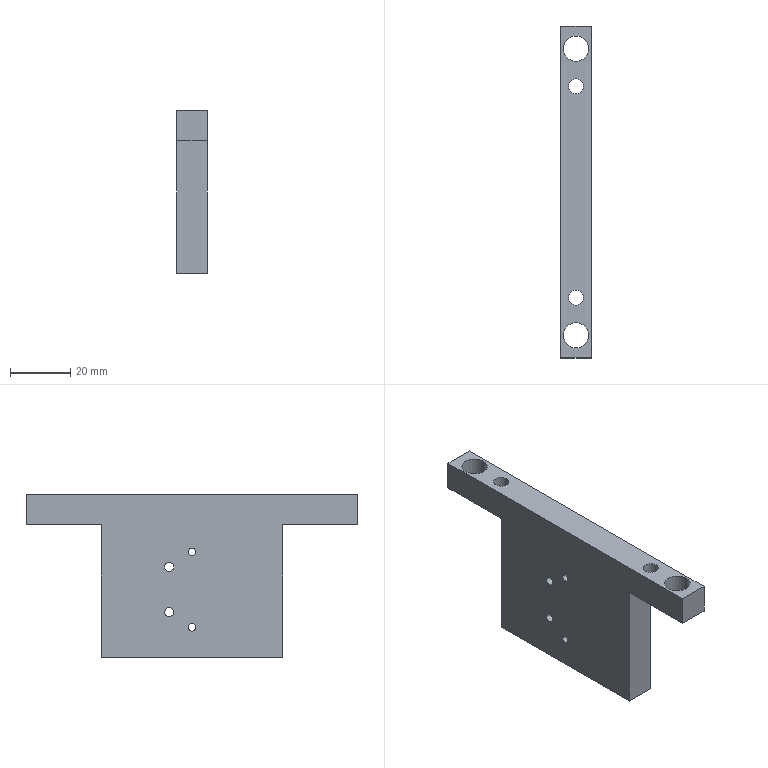Component | SolidWorks | JQ-2-0-002-1 | 1 solid | 34 faces | box 10 x 110 x 54 mm | volume 35051 mm3 | cylinder 20 | plane 10 | cone 4 | commonest cylinder face diameters 5 x8 3 x4 8.4 x4 2.5 x4
STEP:
#1=CARTESIAN_POINT('',(-13.467,1.509,-0.03421));
#2=VERTEX_POINT('',#1);
#3=CARTESIAN_POINT('',(-13.467,1.391,-0.03421));
#4=VERTEX_POINT('',#3);
#5=CARTESIAN_POINT('',(-13.467,1.45,-0.03421));
#6=DIRECTION('',(-1.,0.,0.));
#7=DIRECTION('',(0.,-1.,0.));
#8=AXIS2_PLACEMENT_3D('',#5,#6,#7);
#9=CIRCLE('',#8,0.05906);
#10=EDGE_CURVE('',#2,#4,#9,.T.);
#11=ORIENTED_EDGE('',*,*,#10,.T.);
#12=CARTESIAN_POINT('',(-13.073,1.391,-0.03421));
#13=VERTEX_POINT('',#12);
#14=CARTESIAN_POINT('',(-13.467,1.391,-0.03421));
#15=DIRECTION('',(1.,-0.,-0.));
#16=VECTOR('',#15,39.37);
#17=LINE('',#14,#16);
#18=EDGE_CURVE('',#4,#13,#17,.T.);
#19=ORIENTED_EDGE('',*,*,#18,.T.);
#20=CARTESIAN_POINT('',(-13.073,1.509,-0.03421));
#21=VERTEX_POINT('',#20);
#22=CARTESIAN_POINT('',(-13.073,1.45,-0.03421));
#23=DIRECTION('',(1.,-0.,-0.));
#24=DIRECTION('',(0.,1.,0.));
#25=AXIS2_PLACEMENT_3D('',#22,#23,#24);
#26=CIRCLE('',#25,0.05906);
#27=EDGE_CURVE('',#13,#21,#26,.T.);
#28=ORIENTED_EDGE('',*,*,#27,.T.);
#29=CARTESIAN_POINT('',(-13.467,1.509,-0.03421));
#30=DIRECTION('',(1.,-0.,-0.));
#31=VECTOR('',#30,39.37);
#32=LINE('',#29,#31);
#33=EDGE_CURVE('',#2,#21,#32,.T.);
#34=ORIENTED_EDGE('',*,*,#33,.F.);
#35=EDGE_LOOP('',(#11,#19,#28,#34));
#36=FACE_OUTER_BOUND('',#35,.T.);
#37=CARTESIAN_POINT('',(-13.467,1.45,-0.03421));
#38=DIRECTION('',(1.,-0.,-0.));
#39=DIRECTION('',(0.,1.,0.));
#40=AXIS2_PLACEMENT_3D('',#37,#38,#39);
#41=CYLINDRICAL_SURFACE('',#40,0.05906);
#42=ADVANCED_FACE('',(#36),#41,.F.);
#43=CARTESIAN_POINT('',(-13.467,1.509,0.5563));
#44=VERTEX_POINT('',#43);
#45=CARTESIAN_POINT('',(-13.467,1.391,0.5563));
#46=VERTEX_POINT('',#45);
#47=CARTESIAN_POINT('',(-13.467,1.45,0.5563));
#48=DIRECTION('',(-1.,0.,0.));
#49=DIRECTION('',(0.,-1.,0.));
#50=AXIS2_PLACEMENT_3D('',#47,#48,#49);
#51=CIRCLE('',#50,0.05906);
#52=EDGE_CURVE('',#44,#46,#51,.T.);
#53=ORIENTED_EDGE('',*,*,#52,.T.);
#54=CARTESIAN_POINT('',(-13.073,1.391,0.5563));
#55=VERTEX_POINT('',#54);
#56=CARTESIAN_POINT('',(-13.467,1.391,0.5563));
#57=DIRECTION('',(1.,-0.,-0.));
#58=VECTOR('',#57,39.37);
#59=LINE('',#56,#58);
#60=EDGE_CURVE('',#46,#55,#59,.T.);
#61=ORIENTED_EDGE('',*,*,#60,.T.);
#62=CARTESIAN_POINT('',(-13.073,1.509,0.5563));
#63=VERTEX_POINT('',#62);
#64=CARTESIAN_POINT('',(-13.073,1.45,0.5563));
#65=DIRECTION('',(1.,-0.,-0.));
#66=DIRECTION('',(0.,1.,0.));
#67=AXIS2_PLACEMENT_3D('',#64,#65,#66);
#68=CIRCLE('',#67,0.05906);
#69=EDGE_CURVE('',#55,#63,#68,.T.);
#70=ORIENTED_EDGE('',*,*,#69,.T.);
#71=CARTESIAN_POINT('',(-13.467,1.509,0.5563));
#72=DIRECTION('',(1.,-0.,-0.));
#73=VECTOR('',#72,39.37);
#74=LINE('',#71,#73);
#75=EDGE_CURVE('',#44,#63,#74,.T.);
#76=ORIENTED_EDGE('',*,*,#75,.F.);
#77=EDGE_LOOP('',(#53,#61,#70,#76));
#78=FACE_OUTER_BOUND('',#77,.T.);
#79=CARTESIAN_POINT('',(-13.467,1.45,0.5563));
#80=DIRECTION('',(1.,-0.,-0.));
#81=DIRECTION('',(0.,1.,0.));
#82=AXIS2_PLACEMENT_3D('',#79,#80,#81);
#83=CYLINDRICAL_SURFACE('',#82,0.05906);
#84=ADVANCED_FACE('',(#78),#83,.F.);
#85=CARTESIAN_POINT('',(-13.368,-0.2229,1.108));
#86=VERTEX_POINT('',#85);
#87=CARTESIAN_POINT('',(-13.172,-0.2229,1.108));
#88=VERTEX_POINT('',#87);
#89=CARTESIAN_POINT('',(-13.27,-0.2229,1.108));
#90=DIRECTION('',(0.,-0.,1.));
#91=DIRECTION('',(-1.,0.,0.));
#92=AXIS2_PLACEMENT_3D('',#89,#90,#91);
#93=CIRCLE('',#92,0.09843);
#94=EDGE_CURVE('',#86,#88,#93,.T.);
#95=ORIENTED_EDGE('',*,*,#94,.F.);
#96=CARTESIAN_POINT('',(-13.368,-0.2229,1.501));
#97=VERTEX_POINT('',#96);
#98=CARTESIAN_POINT('',(-13.368,-0.2229,-0.6248));
#99=DIRECTION('',(0.,-0.,1.));
#100=VECTOR('',#99,39.37);
#101=LINE('',#98,#100);
#102=EDGE_CURVE('',#86,#97,#101,.T.);
#103=ORIENTED_EDGE('',*,*,#102,.T.);
#104=CARTESIAN_POINT('',(-13.172,-0.2229,1.501));
#105=VERTEX_POINT('',#104);
#106=CARTESIAN_POINT('',(-13.27,-0.2229,1.501));
#107=DIRECTION('',(0.,-0.,1.));
#108=DIRECTION('',(1.,-0.,0.));
#109=AXIS2_PLACEMENT_3D('',#106,#107,#108);
#110=CIRCLE('',#109,0.09843);
#111=EDGE_CURVE('',#97,#105,#110,.T.);
#112=ORIENTED_EDGE('',*,*,#111,.T.);
#113=CARTESIAN_POINT('',(-13.172,-0.2229,-0.6248));
#114=DIRECTION('',(0.,-0.,1.));
#115=VECTOR('',#114,39.37);
#116=LINE('',#113,#115);
#117=EDGE_CURVE('',#88,#105,#116,.T.);
#118=ORIENTED_EDGE('',*,*,#117,.F.);
#119=EDGE_LOOP('',(#95,#103,#112,#118));
#120=FACE_OUTER_BOUND('',#119,.T.);
#121=CARTESIAN_POINT('',(-13.27,-0.2229,-0.6248));
#122=DIRECTION('',(0.,-0.,1.));
#123=DIRECTION('',(1.,-0.,0.));
#124=AXIS2_PLACEMENT_3D('',#121,#122,#123);
#125=CYLINDRICAL_SURFACE('',#124,0.09843);
#126=ADVANCED_FACE('',(#120),#125,.F.);
#127=CARTESIAN_POINT('',(-13.368,2.533,1.108));
#128=VERTEX_POINT('',#127);
#129=CARTESIAN_POINT('',(-13.172,2.533,1.108));
#130=VERTEX_POINT('',#129);
#131=CARTESIAN_POINT('',(-13.27,2.533,1.108));
#132=DIRECTION('',(0.,-0.,1.));
#133=DIRECTION('',(0.,1.,0.));
#134=AXIS2_PLACEMENT_3D('',#131,#132,#133);
#135=CIRCLE('',#134,0.09843);
#136=EDGE_CURVE('',#128,#130,#135,.T.);
#137=ORIENTED_EDGE('',*,*,#136,.F.);
#138=CARTESIAN_POINT('',(-13.368,2.533,1.501));
#139=VERTEX_POINT('',#138);
#140=CARTESIAN_POINT('',(-13.368,2.533,-0.6248));
#141=DIRECTION('',(0.,-0.,1.));
#142=VECTOR('',#141,39.37);
#143=LINE('',#140,#142);
#144=EDGE_CURVE('',#128,#139,#143,.T.);
#145=ORIENTED_EDGE('',*,*,#144,.T.);
#146=CARTESIAN_POINT('',(-13.172,2.533,1.501));
#147=VERTEX_POINT('',#146);
#148=CARTESIAN_POINT('',(-13.27,2.533,1.501));
#149=DIRECTION('',(0.,-0.,1.));
#150=DIRECTION('',(1.,0.,0.));
#151=AXIS2_PLACEMENT_3D('',#148,#149,#150);
#152=CIRCLE('',#151,0.09843);
#153=EDGE_CURVE('',#139,#147,#152,.T.);
#154=ORIENTED_EDGE('',*,*,#153,.T.);
#155=CARTESIAN_POINT('',(-13.172,2.533,-0.6248));
#156=DIRECTION('',(0.,-0.,1.));
#157=VECTOR('',#156,39.37);
#158=LINE('',#155,#157);
#159=EDGE_CURVE('',#130,#147,#158,.T.);
#160=ORIENTED_EDGE('',*,*,#159,.F.);
#161=EDGE_LOOP('',(#137,#145,#154,#160));
#162=FACE_OUTER_BOUND('',#161,.T.);
#163=CARTESIAN_POINT('',(-13.27,2.533,-0.6248));
#164=DIRECTION('',(0.,-0.,1.));
#165=DIRECTION('',(1.,0.,0.));
#166=AXIS2_PLACEMENT_3D('',#163,#164,#165);
#167=CYLINDRICAL_SURFACE('',#166,0.09843);
#168=ADVANCED_FACE('',(#162),#167,.F.);
#169=CARTESIAN_POINT('',(-13.435,3.025,1.108));
#170=VERTEX_POINT('',#169);
#171=CARTESIAN_POINT('',(-13.105,3.025,1.108));
#172=VERTEX_POINT('',#171);
#173=CARTESIAN_POINT('',(-13.27,3.025,1.108));
#174=DIRECTION('',(0.,-0.,1.));
#175=DIRECTION('',(0.,1.,0.));
#176=AXIS2_PLACEMENT_3D('',#173,#174,#175);
#177=CIRCLE('',#176,0.1654);
#178=EDGE_CURVE('',#170,#172,#177,.T.);
#179=ORIENTED_EDGE('',*,*,#178,.F.);
#180=CARTESIAN_POINT('',(-13.435,3.025,1.501));
#181=VERTEX_POINT('',#180);
#182=CARTESIAN_POINT('',(-13.435,3.025,-0.6248));
#183=DIRECTION('',(0.,-0.,1.));
#184=VECTOR('',#183,39.37);
#185=LINE('',#182,#184);
#186=EDGE_CURVE('',#170,#181,#185,.T.);
#187=ORIENTED_EDGE('',*,*,#186,.T.);
#188=CARTESIAN_POINT('',(-13.105,3.025,1.501));
#189=VERTEX_POINT('',#188);
#190=CARTESIAN_POINT('',(-13.27,3.025,1.501));
#191=DIRECTION('',(0.,-0.,1.));
#192=DIRECTION('',(1.,0.,0.));
#193=AXIS2_PLACEMENT_3D('',#190,#191,#192);
#194=CIRCLE('',#193,0.1654);
#195=EDGE_CURVE('',#181,#189,#194,.T.);
#196=ORIENTED_EDGE('',*,*,#195,.T.);
#197=CARTESIAN_POINT('',(-13.105,3.025,-0.6248));
#198=DIRECTION('',(0.,-0.,1.));
#199=VECTOR('',#198,39.37);
#200=LINE('',#197,#199);
#201=EDGE_CURVE('',#172,#189,#200,.T.);
#202=ORIENTED_EDGE('',*,*,#201,.F.);
#203=EDGE_LOOP('',(#179,#187,#196,#202));
#204=FACE_OUTER_BOUND('',#203,.T.);
#205=CARTESIAN_POINT('',(-13.27,3.025,-0.6248));
#206=DIRECTION('',(0.,-0.,1.));
#207=DIRECTION('',(1.,0.,0.));
#208=AXIS2_PLACEMENT_3D('',#205,#206,#207);
#209=CYLINDRICAL_SURFACE('',#208,0.1654);
#210=ADVANCED_FACE('',(#204),#209,.F.);
#211=CARTESIAN_POINT('',(-13.435,-0.715,1.108));
#212=VERTEX_POINT('',#211);
#213=CARTESIAN_POINT('',(-13.105,-0.715,1.108));
#214=VERTEX_POINT('',#213);
#215=CARTESIAN_POINT('',(-13.27,-0.715,1.108));
#216=DIRECTION('',(0.,-0.,1.));
#217=DIRECTION('',(-1.,0.,0.));
#218=AXIS2_PLACEMENT_3D('',#215,#216,#217);
#219=CIRCLE('',#218,0.1654);
#220=EDGE_CURVE('',#212,#214,#219,.T.);
#221=ORIENTED_EDGE('',*,*,#220,.F.);
#222=CARTESIAN_POINT('',(-13.435,-0.715,1.501));
#223=VERTEX_POINT('',#222);
#224=CARTESIAN_POINT('',(-13.435,-0.715,-0.6248));
#225=DIRECTION('',(0.,-0.,1.));
#226=VECTOR('',#225,39.37);
#227=LINE('',#224,#226);
#228=EDGE_CURVE('',#212,#223,#227,.T.);
#229=ORIENTED_EDGE('',*,*,#228,.T.);
#230=CARTESIAN_POINT('',(-13.105,-0.715,1.501));
#231=VERTEX_POINT('',#230);
#232=CARTESIAN_POINT('',(-13.27,-0.715,1.501));
#233=DIRECTION('',(0.,-0.,1.));
#234=DIRECTION('',(1.,-0.,0.));
#235=AXIS2_PLACEMENT_3D('',#232,#233,#234);
#236=CIRCLE('',#235,0.1654);
#237=EDGE_CURVE('',#223,#231,#236,.T.);
#238=ORIENTED_EDGE('',*,*,#237,.T.);
#239=CARTESIAN_POINT('',(-13.105,-0.715,-0.6248));
#240=DIRECTION('',(0.,-0.,1.));
#241=VECTOR('',#240,39.37);
#242=LINE('',#239,#241);
#243=EDGE_CURVE('',#214,#231,#242,.T.);
#244=ORIENTED_EDGE('',*,*,#243,.F.);
#245=EDGE_LOOP('',(#221,#229,#238,#244));
#246=FACE_OUTER_BOUND('',#245,.T.);
#247=CARTESIAN_POINT('',(-13.27,-0.715,-0.6248));
#248=DIRECTION('',(0.,-0.,1.));
#249=DIRECTION('',(1.,-0.,0.));
#250=AXIS2_PLACEMENT_3D('',#247,#248,#249);
#251=CYLINDRICAL_SURFACE('',#250,0.1654);
#252=ADVANCED_FACE('',(#246),#251,.F.);
#253=CARTESIAN_POINT('',(-13.172,2.139,-0.03421));
#254=VERTEX_POINT('',#253);
#255=CARTESIAN_POINT('',(-13.368,2.139,-0.03421));
#256=VERTEX_POINT('',#255);
#257=CARTESIAN_POINT('',(-13.27,2.139,-0.03421));
#258=DIRECTION('',(-0.,0.,-1.));
#259=DIRECTION('',(-1.,0.,0.));
#260=AXIS2_PLACEMENT_3D('',#257,#258,#259);
#261=CIRCLE('',#260,0.09843);
#262=EDGE_CURVE('',#254,#256,#261,.T.);
#263=ORIENTED_EDGE('',*,*,#262,.F.);
#264=CARTESIAN_POINT('',(-13.172,2.139,-0.6248));
#265=VERTEX_POINT('',#264);
#266=CARTESIAN_POINT('',(-13.172,2.139,-0.6248));
#267=DIRECTION('',(-0.,0.,-1.));
#268=VECTOR('',#267,39.37);
#269=LINE('',#266,#268);
#270=EDGE_CURVE('',#254,#265,#269,.T.);
#271=ORIENTED_EDGE('',*,*,#270,.T.);
#272=CARTESIAN_POINT('',(-13.368,2.139,-0.6248));
#273=VERTEX_POINT('',#272);
#274=CARTESIAN_POINT('',(-13.27,2.139,-0.6248));
#275=DIRECTION('',(-0.,0.,-1.));
#276=DIRECTION('',(-1.,0.,0.));
#277=AXIS2_PLACEMENT_3D('',#274,#275,#276);
#278=CIRCLE('',#277,0.09843);
#279=EDGE_CURVE('',#265,#273,#278,.T.);
#280=ORIENTED_EDGE('',*,*,#279,.T.);
#281=CARTESIAN_POINT('',(-13.368,2.139,-0.6248));
#282=DIRECTION('',(-0.,0.,-1.));
#283=VECTOR('',#282,39.37);
#284=LINE('',#281,#283);
#285=EDGE_CURVE('',#256,#273,#284,.T.);
#286=ORIENTED_EDGE('',*,*,#285,.F.);
#287=EDGE_LOOP('',(#263,#271,#280,#286));
#288=FACE_OUTER_BOUND('',#287,.T.);
#289=CARTESIAN_POINT('',(-13.27,2.139,-0.6248));
#290=DIRECTION('',(-0.,0.,-1.));
#291=DIRECTION('',(-1.,0.,0.));
#292=AXIS2_PLACEMENT_3D('',#289,#290,#291);
#293=CYLINDRICAL_SURFACE('',#292,0.09843);
#294=ADVANCED_FACE('',(#288),#293,.F.);
#295=CARTESIAN_POINT('',(-13.27,2.139,0.02493));
#296=VERTEX_POINT('',#295);
#297=CARTESIAN_POINT('',(-13.368,2.139,-0.03421));
#298=DIRECTION('',(-0.8572,0.,-0.515));
#299=VECTOR('',#298,39.37);
#300=LINE('',#297,#299);
#301=EDGE_CURVE('',#296,#256,#300,.T.);
#302=ORIENTED_EDGE('',*,*,#301,.F.);
#303=CARTESIAN_POINT('',(-13.172,2.139,-0.03421));
#304=DIRECTION('',(0.8572,-0.,-0.515));
#305=VECTOR('',#304,39.37);
#306=LINE('',#303,#305);
#307=EDGE_CURVE('',#296,#254,#306,.T.);
#308=ORIENTED_EDGE('',*,*,#307,.T.);
#309=ORIENTED_EDGE('',*,*,#262,.T.);
#310=EDGE_LOOP('',(#302,#308,#309));
#311=FACE_OUTER_BOUND('',#310,.T.);
#312=CARTESIAN_POINT('',(-13.27,2.139,-0.03421));
#313=DIRECTION('',(-0.,0.,-1.));
#314=DIRECTION('',(-1.,0.,0.));
#315=AXIS2_PLACEMENT_3D('',#312,#313,#314);
#316=CONICAL_SURFACE('',#315,0.09843,1.03);
#317=ADVANCED_FACE('',(#311),#316,.F.);
#318=CARTESIAN_POINT('',(-13.172,0.1708,-0.03421));
#319=VERTEX_POINT('',#318);
#320=CARTESIAN_POINT('',(-13.368,0.1708,-0.03421));
#321=VERTEX_POINT('',#320);
#322=CARTESIAN_POINT('',(-13.27,0.1708,-0.03421));
#323=DIRECTION('',(-0.,0.,-1.));
#324=DIRECTION('',(-1.,0.,0.));
#325=AXIS2_PLACEMENT_3D('',#322,#323,#324);
#326=CIRCLE('',#325,0.09843);
#327=EDGE_CURVE('',#319,#321,#326,.T.);
#328=ORIENTED_EDGE('',*,*,#327,.F.);
#329=CARTESIAN_POINT('',(-13.172,0.1708,-0.6248));
#330=VERTEX_POINT('',#329);
#331=CARTESIAN_POINT('',(-13.172,0.1708,-0.6248));
#332=DIRECTION('',(-0.,0.,-1.));
#333=VECTOR('',#332,39.37);
#334=LINE('',#331,#333);
#335=EDGE_CURVE('',#319,#330,#334,.T.);
#336=ORIENTED_EDGE('',*,*,#335,.T.);
#337=CARTESIAN_POINT('',(-13.368,0.1708,-0.6248));
#338=VERTEX_POINT('',#337);
#339=CARTESIAN_POINT('',(-13.27,0.1708,-0.6248));
#340=DIRECTION('',(-0.,0.,-1.));
#341=DIRECTION('',(-1.,0.,0.));
#342=AXIS2_PLACEMENT_3D('',#339,#340,#341);
#343=CIRCLE('',#342,0.09843);
#344=EDGE_CURVE('',#330,#338,#343,.T.);
#345=ORIENTED_EDGE('',*,*,#344,.T.);
#346=CARTESIAN_POINT('',(-13.368,0.1708,-0.6248));
#347=DIRECTION('',(-0.,0.,-1.));
#348=VECTOR('',#347,39.37);
#349=LINE('',#346,#348);
#350=EDGE_CURVE('',#321,#338,#349,.T.);
#351=ORIENTED_EDGE('',*,*,#350,.F.);
#352=EDGE_LOOP('',(#328,#336,#345,#351));
#353=FACE_OUTER_BOUND('',#352,.T.);
#354=CARTESIAN_POINT('',(-13.27,0.1708,-0.6248));
#355=DIRECTION('',(-0.,0.,-1.));
#356=DIRECTION('',(-1.,0.,0.));
#357=AXIS2_PLACEMENT_3D('',#354,#355,#356);
#358=CYLINDRICAL_SURFACE('',#357,0.09843);
#359=ADVANCED_FACE('',(#353),#358,.F.);
#360=CARTESIAN_POINT('',(-13.27,0.1708,0.02493));
#361=VERTEX_POINT('',#360);
#362=CARTESIAN_POINT('',(-13.368,0.1708,-0.03421));
#363=DIRECTION('',(-0.8572,0.,-0.515));
#364=VECTOR('',#363,39.37);
#365=LINE('',#362,#364);
#366=EDGE_CURVE('',#361,#321,#365,.T.);
#367=ORIENTED_EDGE('',*,*,#366,.F.);
#368=CARTESIAN_POINT('',(-13.172,0.1708,-0.03421));
#369=DIRECTION('',(0.8572,-0.,-0.515));
#370=VECTOR('',#369,39.37);
#371=LINE('',#368,#370);
#372=EDGE_CURVE('',#361,#319,#371,.T.);
#373=ORIENTED_EDGE('',*,*,#372,.T.);
#374=ORIENTED_EDGE('',*,*,#327,.T.);
#375=EDGE_LOOP('',(#367,#373,#374));
#376=FACE_OUTER_BOUND('',#375,.T.);
#377=CARTESIAN_POINT('',(-13.27,0.1708,-0.03421));
#378=DIRECTION('',(-0.,0.,-1.));
#379=DIRECTION('',(-1.,0.,0.));
#380=AXIS2_PLACEMENT_3D('',#377,#378,#379);
#381=CONICAL_SURFACE('',#380,0.09843,1.03);
#382=ADVANCED_FACE('',(#376),#381,.F.);
#383=CARTESIAN_POINT('',(-13.467,1.106,0.7532));
#384=VERTEX_POINT('',#383);
#385=CARTESIAN_POINT('',(-13.467,1.204,0.7532));
#386=VERTEX_POINT('',#385);
#387=CARTESIAN_POINT('',(-13.467,1.155,0.7532));
#388=DIRECTION('',(1.,-0.,-0.));
#389=DIRECTION('',(0.,1.,0.));
#390=AXIS2_PLACEMENT_3D('',#387,#388,#389);
#391=CIRCLE('',#390,0.04921);
#392=EDGE_CURVE('',#384,#386,#391,.T.);
#393=ORIENTED_EDGE('',*,*,#392,.F.);
#394=CARTESIAN_POINT('',(-13.073,1.106,0.7532));
#395=VERTEX_POINT('',#394);
#396=CARTESIAN_POINT('',(-13.073,1.106,0.7532));
#397=DIRECTION('',(1.,-0.,-0.));
#398=VECTOR('',#397,39.37);
#399=LINE('',#396,#398);
#400=EDGE_CURVE('',#384,#395,#399,.T.);
#401=ORIENTED_EDGE('',*,*,#400,.T.);
#402=CARTESIAN_POINT('',(-13.073,1.204,0.7532));
#403=VERTEX_POINT('',#402);
#404=CARTESIAN_POINT('',(-13.073,1.155,0.7532));
#405=DIRECTION('',(1.,-0.,-0.));
#406=DIRECTION('',(0.,1.,0.));
#407=AXIS2_PLACEMENT_3D('',#404,#405,#406);
#408=CIRCLE('',#407,0.04921);
#409=EDGE_CURVE('',#395,#403,#408,.T.);
#410=ORIENTED_EDGE('',*,*,#409,.T.);
#411=CARTESIAN_POINT('',(-13.073,1.204,0.7532));
#412=DIRECTION('',(1.,-0.,-0.));
#413=VECTOR('',#412,39.37);
#414=LINE('',#411,#413);
#415=EDGE_CURVE('',#386,#403,#414,.T.);
#416=ORIENTED_EDGE('',*,*,#415,.F.);
#417=EDGE_LOOP('',(#393,#401,#410,#416));
#418=FACE_OUTER_BOUND('',#417,.T.);
#419=CARTESIAN_POINT('',(-13.073,1.155,0.7532));
#420=DIRECTION('',(1.,-0.,-0.));
#421=DIRECTION('',(0.,1.,0.));
#422=AXIS2_PLACEMENT_3D('',#419,#420,#421);
#423=CYLINDRICAL_SURFACE('',#422,0.04921);
#424=ADVANCED_FACE('',(#418),#423,.F.);
#425=CARTESIAN_POINT('',(-13.467,1.106,-0.2311));
#426=VERTEX_POINT('',#425);
#427=CARTESIAN_POINT('',(-13.467,1.204,-0.2311));
#428=VERTEX_POINT('',#427);
#429=CARTESIAN_POINT('',(-13.467,1.155,-0.2311));
#430=DIRECTION('',(1.,-0.,-0.));
#431=DIRECTION('',(0.,1.,0.));
#432=AXIS2_PLACEMENT_3D('',#429,#430,#431);
#433=CIRCLE('',#432,0.04921);
#434=EDGE_CURVE('',#426,#428,#433,.T.);
#435=ORIENTED_EDGE('',*,*,#434,.F.);
#436=CARTESIAN_POINT('',(-13.073,1.106,-0.2311));
#437=VERTEX_POINT('',#436);
#438=CARTESIAN_POINT('',(-13.073,1.106,-0.2311));
#439=DIRECTION('',(1.,-0.,-0.));
#440=VECTOR('',#439,39.37);
#441=LINE('',#438,#440);
#442=EDGE_CURVE('',#426,#437,#441,.T.);
#443=ORIENTED_EDGE('',*,*,#442,.T.);
#444=CARTESIAN_POINT('',(-13.073,1.204,-0.2311));
#445=VERTEX_POINT('',#444);
#446=CARTESIAN_POINT('',(-13.073,1.155,-0.2311));
#447=DIRECTION('',(1.,-0.,-0.));
#448=DIRECTION('',(0.,1.,0.));
#449=AXIS2_PLACEMENT_3D('',#446,#447,#448);
#450=CIRCLE('',#449,0.04921);
#451=EDGE_CURVE('',#437,#445,#450,.T.);
#452=ORIENTED_EDGE('',*,*,#451,.T.);
#453=CARTESIAN_POINT('',(-13.073,1.204,-0.2311));
#454=DIRECTION('',(1.,-0.,-0.));
#455=VECTOR('',#454,39.37);
#456=LINE('',#453,#455);
#457=EDGE_CURVE('',#428,#445,#456,.T.);
#458=ORIENTED_EDGE('',*,*,#457,.F.);
#459=EDGE_LOOP('',(#435,#443,#452,#458));
#460=FACE_OUTER_BOUND('',#459,.T.);
#461=CARTESIAN_POINT('',(-13.073,1.155,-0.2311));
#462=DIRECTION('',(1.,-0.,-0.));
#463=DIRECTION('',(0.,1.,0.));
#464=AXIS2_PLACEMENT_3D('',#461,#462,#463);
#465=CYLINDRICAL_SURFACE('',#464,0.04921);
#466=ADVANCED_FACE('',(#460),#465,.F.);
#467=CARTESIAN_POINT('',(-13.467,-0.02602,1.108));
#468=VERTEX_POINT('',#467);
#469=CARTESIAN_POINT('',(-13.073,-0.02602,1.108));
#470=VERTEX_POINT('',#469);
#471=CARTESIAN_POINT('',(-14.527,-0.02602,1.108));
#472=DIRECTION('',(1.,-0.,-0.));
#473=VECTOR('',#472,39.37);
#474=LINE('',#471,#473);
#475=EDGE_CURVE('',#468,#470,#474,.T.);
#476=ORIENTED_EDGE('',*,*,#475,.F.);
#477=CARTESIAN_POINT('',(-13.467,-0.02602,-0.6248));
#478=VERTEX_POINT('',#477);
#479=CARTESIAN_POINT('',(-13.467,-0.02602,-0.6248));
#480=DIRECTION('',(-0.,0.,-1.));
#481=VECTOR('',#480,39.37);
#482=LINE('',#479,#481);
#483=EDGE_CURVE('',#468,#478,#482,.T.);
#484=ORIENTED_EDGE('',*,*,#483,.T.);
#485=CARTESIAN_POINT('',(-13.073,-0.02602,-0.6248));
#486=VERTEX_POINT('',#485);
#487=CARTESIAN_POINT('',(-13.073,-0.02602,-0.6248));
#488=DIRECTION('',(-1.,0.,0.));
#489=VECTOR('',#488,39.37);
#490=LINE('',#487,#489);
#491=EDGE_CURVE('',#486,#478,#490,.T.);
#492=ORIENTED_EDGE('',*,*,#491,.F.);
#493=CARTESIAN_POINT('',(-13.073,-0.02602,-0.6248));
#494=DIRECTION('',(-0.,0.,-1.));
#495=VECTOR('',#494,39.37);
#496=LINE('',#493,#495);
#497=EDGE_CURVE('',#470,#486,#496,.T.);
#498=ORIENTED_EDGE('',*,*,#497,.F.);
#499=EDGE_LOOP('',(#476,#484,#492,#498));
#500=FACE_OUTER_BOUND('',#499,.T.);
#501=CARTESIAN_POINT('',(-13.073,-0.02602,-0.6248));
#502=DIRECTION('',(0.,1.,0.));
#503=DIRECTION('',(-1.,0.,0.));
#504=AXIS2_PLACEMENT_3D('',#501,#502,#503);
#505=PLANE('',#504);
#506=ADVANCED_FACE('',(#500),#505,.F.);
#507=CARTESIAN_POINT('',(-13.27,2.139,-0.6248));
#508=DIRECTION('',(-0.,0.,-1.));
#509=DIRECTION('',(-1.,0.,0.));
#510=AXIS2_PLACEMENT_3D('',#507,#508,#509);
#511=CIRCLE('',#510,0.09843);
#512=EDGE_CURVE('',#273,#265,#511,.T.);
#513=ORIENTED_EDGE('',*,*,#512,.F.);
#514=ORIENTED_EDGE('',*,*,#279,.F.);
#515=EDGE_LOOP('',(#513,#514));
#516=FACE_BOUND('',#515,.T.);
#517=CARTESIAN_POINT('',(-13.27,0.1708,-0.6248));
#518=DIRECTION('',(-0.,0.,-1.));
#519=DIRECTION('',(-1.,0.,0.));
#520=AXIS2_PLACEMENT_3D('',#517,#518,#519);
#521=CIRCLE('',#520,0.09843);
#522=EDGE_CURVE('',#338,#330,#521,.T.);
#523=ORIENTED_EDGE('',*,*,#522,.F.);
#524=ORIENTED_EDGE('',*,*,#344,.F.);
#525=EDGE_LOOP('',(#523,#524));
#526=FACE_BOUND('',#525,.T.);
#527=CARTESIAN_POINT('',(-13.467,2.336,-0.6248));
#528=VERTEX_POINT('',#527);
#529=CARTESIAN_POINT('',(-13.467,-0.02602,-0.6248));
#530=DIRECTION('',(0.,1.,0.));
#531=VECTOR('',#530,39.37);
#532=LINE('',#529,#531);
#533=EDGE_CURVE('',#478,#528,#532,.T.);
#534=ORIENTED_EDGE('',*,*,#533,.T.);
#535=CARTESIAN_POINT('',(-13.073,2.336,-0.6248));
#536=VERTEX_POINT('',#535);
#537=CARTESIAN_POINT('',(-13.073,2.336,-0.6248));
#538=DIRECTION('',(-1.,0.,0.));
#539=VECTOR('',#538,39.37);
#540=LINE('',#537,#539);
#541=EDGE_CURVE('',#536,#528,#540,.T.);
#542=ORIENTED_EDGE('',*,*,#541,.F.);
#543=CARTESIAN_POINT('',(-13.073,-0.02602,-0.6248));
#544=DIRECTION('',(0.,1.,0.));
#545=VECTOR('',#544,39.37);
#546=LINE('',#543,#545);
#547=EDGE_CURVE('',#486,#536,#546,.T.);
#548=ORIENTED_EDGE('',*,*,#547,.F.);
#549=ORIENTED_EDGE('',*,*,#491,.T.);
#550=EDGE_LOOP('',(#534,#542,#548,#549));
#551=FACE_OUTER_BOUND('',#550,.T.);
#552=CARTESIAN_POINT('',(-13.073,-0.02602,-0.6248));
#553=DIRECTION('',(0.,-0.,1.));
#554=DIRECTION('',(1.,-0.,-0.));
#555=AXIS2_PLACEMENT_3D('',#552,#553,#554);
#556=PLANE('',#555);
#557=ADVANCED_FACE('',(#516,#526,#551),#556,.F.);
#558=CARTESIAN_POINT('',(-13.467,2.336,1.108));
#559=VERTEX_POINT('',#558);
#560=CARTESIAN_POINT('',(-13.467,2.336,-0.6248));
#561=DIRECTION('',(0.,-0.,1.));
#562=VECTOR('',#561,39.37);
#563=LINE('',#560,#562);
#564=EDGE_CURVE('',#528,#559,#563,.T.);
#565=ORIENTED_EDGE('',*,*,#564,.T.);
#566=CARTESIAN_POINT('',(-13.073,2.336,1.108));
#567=VERTEX_POINT('',#566);
#568=CARTESIAN_POINT('',(-14.527,2.336,1.108));
#569=DIRECTION('',(1.,-0.,-0.));
#570=VECTOR('',#569,39.37);
#571=LINE('',#568,#570);
#572=EDGE_CURVE('',#559,#567,#571,.T.);
#573=ORIENTED_EDGE('',*,*,#572,.T.);
#574=CARTESIAN_POINT('',(-13.073,2.336,-0.6248));
#575=DIRECTION('',(0.,-0.,1.));
#576=VECTOR('',#575,39.37);
#577=LINE('',#574,#576);
#578=EDGE_CURVE('',#536,#567,#577,.T.);
#579=ORIENTED_EDGE('',*,*,#578,.F.);
#580=ORIENTED_EDGE('',*,*,#541,.T.);
#581=EDGE_LOOP('',(#565,#573,#579,#580));
#582=FACE_OUTER_BOUND('',#581,.T.);
#583=CARTESIAN_POINT('',(-13.073,2.336,-0.6248));
#584=DIRECTION('',(-0.,-1.,-0.));
#585=DIRECTION('',(1.,-0.,-0.));
#586=AXIS2_PLACEMENT_3D('',#583,#584,#585);
#587=PLANE('',#586);
#588=ADVANCED_FACE('',(#582),#587,.F.);
#589=CARTESIAN_POINT('',(-13.27,-0.2229,1.501));
#590=DIRECTION('',(0.,-0.,1.));
#591=DIRECTION('',(1.,-0.,0.));
#592=AXIS2_PLACEMENT_3D('',#589,#590,#591);
#593=CIRCLE('',#592,0.09843);
#594=EDGE_CURVE('',#105,#97,#593,.T.);
#595=ORIENTED_EDGE('',*,*,#594,.F.);
#596=ORIENTED_EDGE('',*,*,#111,.F.);
#597=EDGE_LOOP('',(#595,#596));
#598=FACE_BOUND('',#597,.T.);
#599=CARTESIAN_POINT('',(-13.27,2.533,1.501));
#600=DIRECTION('',(0.,-0.,1.));
#601=DIRECTION('',(1.,0.,0.));
#602=AXIS2_PLACEMENT_3D('',#599,#600,#601);
#603=CIRCLE('',#602,0.09843);
#604=EDGE_CURVE('',#147,#139,#603,.T.);
#605=ORIENTED_EDGE('',*,*,#604,.F.);
#606=ORIENTED_EDGE('',*,*,#153,.F.);
#607=EDGE_LOOP('',(#605,#606));
#608=FACE_BOUND('',#607,.T.);
#609=CARTESIAN_POINT('',(-13.27,3.025,1.501));
#610=DIRECTION('',(0.,-0.,1.));
#611=DIRECTION('',(1.,0.,0.));
#612=AXIS2_PLACEMENT_3D('',#609,#610,#611);
#613=CIRCLE('',#612,0.1654);
#614=EDGE_CURVE('',#189,#181,#613,.T.);
#615=ORIENTED_EDGE('',*,*,#614,.F.);
#616=ORIENTED_EDGE('',*,*,#195,.F.);
#617=EDGE_LOOP('',(#615,#616));
#618=FACE_BOUND('',#617,.T.);
#619=CARTESIAN_POINT('',(-13.27,-0.715,1.501));
#620=DIRECTION('',(0.,-0.,1.));
#621=DIRECTION('',(1.,-0.,0.));
#622=AXIS2_PLACEMENT_3D('',#619,#620,#621);
#623=CIRCLE('',#622,0.1654);
#624=EDGE_CURVE('',#231,#223,#623,.T.);
#625=ORIENTED_EDGE('',*,*,#624,.F.);
#626=ORIENTED_EDGE('',*,*,#237,.F.);
#627=EDGE_LOOP('',(#625,#626));
#628=FACE_BOUND('',#627,.T.);
#629=CARTESIAN_POINT('',(-13.467,3.32,1.501));
#630=VERTEX_POINT('',#629);
#631=CARTESIAN_POINT('',(-13.467,-1.01,1.501));
#632=VERTEX_POINT('',#631);
#633=CARTESIAN_POINT('',(-13.467,-0.02602,1.501));
#634=DIRECTION('',(-0.,-1.,-0.));
#635=VECTOR('',#634,39.37);
#636=LINE('',#633,#635);
#637=EDGE_CURVE('',#630,#632,#636,.T.);
#638=ORIENTED_EDGE('',*,*,#637,.T.);
#639=CARTESIAN_POINT('',(-13.073,-1.01,1.501));
#640=VERTEX_POINT('',#639);
#641=CARTESIAN_POINT('',(-14.527,-1.01,1.501));
#642=DIRECTION('',(1.,-0.,-0.));
#643=VECTOR('',#642,39.37);
#644=LINE('',#641,#643);
#645=EDGE_CURVE('',#632,#640,#644,.T.);
#646=ORIENTED_EDGE('',*,*,#645,.T.);
#647=CARTESIAN_POINT('',(-13.073,3.32,1.501));
#648=VERTEX_POINT('',#647);
#649=CARTESIAN_POINT('',(-13.073,-0.02602,1.501));
#650=DIRECTION('',(-0.,-1.,-0.));
#651=VECTOR('',#650,39.37);
#652=LINE('',#649,#651);
#653=EDGE_CURVE('',#648,#640,#652,.T.);
#654=ORIENTED_EDGE('',*,*,#653,.F.);
#655=CARTESIAN_POINT('',(-14.527,3.32,1.501));
#656=DIRECTION('',(1.,-0.,-0.));
#657=VECTOR('',#656,39.37);
#658=LINE('',#655,#657);
#659=EDGE_CURVE('',#630,#648,#658,.T.);
#660=ORIENTED_EDGE('',*,*,#659,.F.);
#661=EDGE_LOOP('',(#638,#646,#654,#660));
#662=FACE_OUTER_BOUND('',#661,.T.);
#663=CARTESIAN_POINT('',(-13.073,-0.02602,1.501));
#664=DIRECTION('',(-0.,0.,-1.));
#665=DIRECTION('',(-1.,0.,0.));
#666=AXIS2_PLACEMENT_3D('',#663,#664,#665);
#667=PLANE('',#666);
#668=ADVANCED_FACE('',(#598,#608,#618,#628,#662),#667,.F.);
#669=CARTESIAN_POINT('',(-13.073,1.45,-0.03421));
#670=DIRECTION('',(1.,-0.,-0.));
#671=DIRECTION('',(0.,1.,0.));
#672=AXIS2_PLACEMENT_3D('',#669,#670,#671);
#673=CIRCLE('',#672,0.05906);
#674=EDGE_CURVE('',#21,#13,#673,.T.);
#675=ORIENTED_EDGE('',*,*,#674,.F.);
#676=ORIENTED_EDGE('',*,*,#27,.F.);
#677=EDGE_LOOP('',(#675,#676));
#678=FACE_BOUND('',#677,.T.);
#679=CARTESIAN_POINT('',(-13.073,1.45,0.5563));
#680=DIRECTION('',(1.,-0.,-0.));
#681=DIRECTION('',(0.,1.,0.));
#682=AXIS2_PLACEMENT_3D('',#679,#680,#681);
#683=CIRCLE('',#682,0.05906);
#684=EDGE_CURVE('',#63,#55,#683,.T.);
#685=ORIENTED_EDGE('',*,*,#684,.F.);
#686=ORIENTED_EDGE('',*,*,#69,.F.);
#687=EDGE_LOOP('',(#685,#686));
#688=FACE_BOUND('',#687,.T.);
#689=CARTESIAN_POINT('',(-13.073,1.155,0.7532));
#690=DIRECTION('',(1.,-0.,-0.));
#691=DIRECTION('',(0.,1.,0.));
#692=AXIS2_PLACEMENT_3D('',#689,#690,#691);
#693=CIRCLE('',#692,0.04921);
#694=EDGE_CURVE('',#403,#395,#693,.T.);
#695=ORIENTED_EDGE('',*,*,#694,.F.);
#696=ORIENTED_EDGE('',*,*,#409,.F.);
#697=EDGE_LOOP('',(#695,#696));
#698=FACE_BOUND('',#697,.T.);
#699=CARTESIAN_POINT('',(-13.073,1.155,-0.2311));
#700=DIRECTION('',(1.,-0.,-0.));
#701=DIRECTION('',(0.,1.,0.));
#702=AXIS2_PLACEMENT_3D('',#699,#700,#701);
#703=CIRCLE('',#702,0.04921);
#704=EDGE_CURVE('',#445,#437,#703,.T.);
#705=ORIENTED_EDGE('',*,*,#704,.F.);
#706=ORIENTED_EDGE('',*,*,#451,.F.);
#707=EDGE_LOOP('',(#705,#706));
#708=FACE_BOUND('',#707,.T.);
#709=ORIENTED_EDGE('',*,*,#653,.T.);
#710=CARTESIAN_POINT('',(-13.073,-1.01,1.108));
#711=VERTEX_POINT('',#710);
#712=CARTESIAN_POINT('',(-13.073,-1.01,1.501));
#713=DIRECTION('',(-0.,0.,-1.));
#714=VECTOR('',#713,39.37);
#715=LINE('',#712,#714);
#716=EDGE_CURVE('',#640,#711,#715,.T.);
#717=ORIENTED_EDGE('',*,*,#716,.T.);
#718=CARTESIAN_POINT('',(-13.073,-0.02602,1.108));
#719=DIRECTION('',(0.,1.,0.));
#720=VECTOR('',#719,39.37);
#721=LINE('',#718,#720);
#722=EDGE_CURVE('',#711,#470,#721,.T.);
#723=ORIENTED_EDGE('',*,*,#722,.T.);
#724=ORIENTED_EDGE('',*,*,#497,.T.);
#725=ORIENTED_EDGE('',*,*,#547,.T.);
#726=ORIENTED_EDGE('',*,*,#578,.T.);
#727=CARTESIAN_POINT('',(-13.073,3.32,1.108));
#728=VERTEX_POINT('',#727);
#729=CARTESIAN_POINT('',(-13.073,2.336,1.108));
#730=DIRECTION('',(0.,1.,0.));
#731=VECTOR('',#730,39.37);
#732=LINE('',#729,#731);
#733=EDGE_CURVE('',#567,#728,#732,.T.);
#734=ORIENTED_EDGE('',*,*,#733,.T.);
#735=CARTESIAN_POINT('',(-13.073,3.32,1.501));
#736=DIRECTION('',(0.,0.,1.));
#737=VECTOR('',#736,39.37);
#738=LINE('',#735,#737);
#739=EDGE_CURVE('',#728,#648,#738,.T.);
#740=ORIENTED_EDGE('',*,*,#739,.T.);
#741=EDGE_LOOP('',(#709,#717,#723,#724,#725,#726,#734,#740));
#742=FACE_OUTER_BOUND('',#741,.T.);
#743=CARTESIAN_POINT('',(-13.073,-0.02602,1.501));
#744=DIRECTION('',(-1.,0.,0.));
#745=DIRECTION('',(-0.,-1.,-0.));
#746=AXIS2_PLACEMENT_3D('',#743,#744,#745);
#747=PLANE('',#746);
#748=ADVANCED_FACE('',(#678,#688,#698,#708,#742),#747,.F.);
#749=ORIENTED_EDGE('',*,*,#10,.F.);
#750=CARTESIAN_POINT('',(-13.467,1.45,-0.03421));
#751=DIRECTION('',(-1.,0.,0.));
#752=DIRECTION('',(0.,-1.,0.));
#753=AXIS2_PLACEMENT_3D('',#750,#751,#752);
#754=CIRCLE('',#753,0.05906);
#755=EDGE_CURVE('',#4,#2,#754,.T.);
#756=ORIENTED_EDGE('',*,*,#755,.F.);
#757=EDGE_LOOP('',(#749,#756));
#758=FACE_BOUND('',#757,.T.);
#759=ORIENTED_EDGE('',*,*,#52,.F.);
#760=CARTESIAN_POINT('',(-13.467,1.45,0.5563));
#761=DIRECTION('',(-1.,0.,0.));
#762=DIRECTION('',(0.,-1.,0.));
#763=AXIS2_PLACEMENT_3D('',#760,#761,#762);
#764=CIRCLE('',#763,0.05906);
#765=EDGE_CURVE('',#46,#44,#764,.T.);
#766=ORIENTED_EDGE('',*,*,#765,.F.);
#767=EDGE_LOOP('',(#759,#766));
#768=FACE_BOUND('',#767,.T.);
#769=CARTESIAN_POINT('',(-13.467,1.155,0.7532));
#770=DIRECTION('',(1.,-0.,-0.));
#771=DIRECTION('',(0.,1.,0.));
#772=AXIS2_PLACEMENT_3D('',#769,#770,#771);
#773=CIRCLE('',#772,0.04921);
#774=EDGE_CURVE('',#386,#384,#773,.T.);
#775=ORIENTED_EDGE('',*,*,#774,.T.);
#776=ORIENTED_EDGE('',*,*,#392,.T.);
#777=EDGE_LOOP('',(#775,#776));
#778=FACE_BOUND('',#777,.T.);
#779=CARTESIAN_POINT('',(-13.467,1.155,-0.2311));
#780=DIRECTION('',(1.,-0.,-0.));
#781=DIRECTION('',(0.,1.,0.));
#782=AXIS2_PLACEMENT_3D('',#779,#780,#781);
#783=CIRCLE('',#782,0.04921);
#784=EDGE_CURVE('',#428,#426,#783,.T.);
#785=ORIENTED_EDGE('',*,*,#784,.T.);
#786=ORIENTED_EDGE('',*,*,#434,.T.);
#787=EDGE_LOOP('',(#785,#786));
#788=FACE_BOUND('',#787,.T.);
#789=ORIENTED_EDGE('',*,*,#483,.F.);
#790=CARTESIAN_POINT('',(-13.467,-1.01,1.108));
#791=VERTEX_POINT('',#790);
#792=CARTESIAN_POINT('',(-13.467,-0.02602,1.108));
#793=DIRECTION('',(0.,1.,0.));
#794=VECTOR('',#793,39.37);
#795=LINE('',#792,#794);
#796=EDGE_CURVE('',#791,#468,#795,.T.);
#797=ORIENTED_EDGE('',*,*,#796,.F.);
#798=CARTESIAN_POINT('',(-13.467,-1.01,1.501));
#799=DIRECTION('',(-0.,0.,-1.));
#800=VECTOR('',#799,39.37);
#801=LINE('',#798,#800);
#802=EDGE_CURVE('',#632,#791,#801,.T.);
#803=ORIENTED_EDGE('',*,*,#802,.F.);
#804=ORIENTED_EDGE('',*,*,#637,.F.);
#805=CARTESIAN_POINT('',(-13.467,3.32,1.108));
#806=VERTEX_POINT('',#805);
#807=CARTESIAN_POINT('',(-13.467,3.32,1.501));
#808=DIRECTION('',(0.,0.,1.));
#809=VECTOR('',#808,39.37);
#810=LINE('',#807,#809);
#811=EDGE_CURVE('',#806,#630,#810,.T.);
#812=ORIENTED_EDGE('',*,*,#811,.F.);
#813=CARTESIAN_POINT('',(-13.467,2.336,1.108));
#814=DIRECTION('',(0.,1.,0.));
#815=VECTOR('',#814,39.37);
#816=LINE('',#813,#815);
#817=EDGE_CURVE('',#559,#806,#816,.T.);
#818=ORIENTED_EDGE('',*,*,#817,.F.);
#819=ORIENTED_EDGE('',*,*,#564,.F.);
#820=ORIENTED_EDGE('',*,*,#533,.F.);
#821=EDGE_LOOP('',(#789,#797,#803,#804,#812,#818,#819,#820));
#822=FACE_OUTER_BOUND('',#821,.T.);
#823=CARTESIAN_POINT('',(-13.467,-0.02602,1.501));
#824=DIRECTION('',(-1.,0.,0.));
#825=DIRECTION('',(-0.,-1.,-0.));
#826=AXIS2_PLACEMENT_3D('',#823,#824,#825);
#827=PLANE('',#826);
#828=ADVANCED_FACE('',(#758,#768,#778,#788,#822),#827,.T.);
#829=ORIENTED_EDGE('',*,*,#442,.F.);
#830=ORIENTED_EDGE('',*,*,#784,.F.);
#831=ORIENTED_EDGE('',*,*,#457,.T.);
#832=ORIENTED_EDGE('',*,*,#704,.T.);
#833=EDGE_LOOP('',(#829,#830,#831,#832));
#834=FACE_OUTER_BOUND('',#833,.T.);
#835=CARTESIAN_POINT('',(-13.073,1.155,-0.2311));
#836=DIRECTION('',(1.,-0.,-0.));
#837=DIRECTION('',(0.,1.,0.));
#838=AXIS2_PLACEMENT_3D('',#835,#836,#837);
#839=CYLINDRICAL_SURFACE('',#838,0.04921);
#840=ADVANCED_FACE('',(#834),#839,.F.);
#841=ORIENTED_EDGE('',*,*,#400,.F.);
#842=ORIENTED_EDGE('',*,*,#774,.F.);
#843=ORIENTED_EDGE('',*,*,#415,.T.);
#844=ORIENTED_EDGE('',*,*,#694,.T.);
#845=EDGE_LOOP('',(#841,#842,#843,#844));
#846=FACE_OUTER_BOUND('',#845,.T.);
#847=CARTESIAN_POINT('',(-13.073,1.155,0.7532));
#848=DIRECTION('',(1.,-0.,-0.));
#849=DIRECTION('',(0.,1.,0.));
#850=AXIS2_PLACEMENT_3D('',#847,#848,#849);
#851=CYLINDRICAL_SURFACE('',#850,0.04921);
#852=ADVANCED_FACE('',(#846),#851,.F.);
#853=ORIENTED_EDGE('',*,*,#372,.F.);
#854=ORIENTED_EDGE('',*,*,#366,.T.);
#855=CARTESIAN_POINT('',(-13.27,0.1708,-0.03421));
#856=DIRECTION('',(-0.,0.,-1.));
#857=DIRECTION('',(-1.,0.,0.));
#858=AXIS2_PLACEMENT_3D('',#855,#856,#857);
#859=CIRCLE('',#858,0.09843);
#860=EDGE_CURVE('',#321,#319,#859,.T.);
#861=ORIENTED_EDGE('',*,*,#860,.T.);
#862=EDGE_LOOP('',(#853,#854,#861));
#863=FACE_OUTER_BOUND('',#862,.T.);
#864=CARTESIAN_POINT('',(-13.27,0.1708,-0.03421));
#865=DIRECTION('',(-0.,0.,-1.));
#866=DIRECTION('',(-1.,0.,0.));
#867=AXIS2_PLACEMENT_3D('',#864,#865,#866);
#868=CONICAL_SURFACE('',#867,0.09843,1.03);
#869=ADVANCED_FACE('',(#863),#868,.F.);
#870=ORIENTED_EDGE('',*,*,#335,.F.);
#871=ORIENTED_EDGE('',*,*,#860,.F.);
#872=ORIENTED_EDGE('',*,*,#350,.T.);
#873=ORIENTED_EDGE('',*,*,#522,.T.);
#874=EDGE_LOOP('',(#870,#871,#872,#873));
#875=FACE_OUTER_BOUND('',#874,.T.);
#876=CARTESIAN_POINT('',(-13.27,0.1708,-0.6248));
#877=DIRECTION('',(-0.,0.,-1.));
#878=DIRECTION('',(-1.,0.,0.));
#879=AXIS2_PLACEMENT_3D('',#876,#877,#878);
#880=CYLINDRICAL_SURFACE('',#879,0.09843);
#881=ADVANCED_FACE('',(#875),#880,.F.);
#882=ORIENTED_EDGE('',*,*,#307,.F.);
#883=ORIENTED_EDGE('',*,*,#301,.T.);
#884=CARTESIAN_POINT('',(-13.27,2.139,-0.03421));
#885=DIRECTION('',(-0.,0.,-1.));
#886=DIRECTION('',(-1.,0.,0.));
#887=AXIS2_PLACEMENT_3D('',#884,#885,#886);
#888=CIRCLE('',#887,0.09843);
#889=EDGE_CURVE('',#256,#254,#888,.T.);
#890=ORIENTED_EDGE('',*,*,#889,.T.);
#891=EDGE_LOOP('',(#882,#883,#890));
#892=FACE_OUTER_BOUND('',#891,.T.);
#893=CARTESIAN_POINT('',(-13.27,2.139,-0.03421));
#894=DIRECTION('',(-0.,0.,-1.));
#895=DIRECTION('',(-1.,0.,0.));
#896=AXIS2_PLACEMENT_3D('',#893,#894,#895);
#897=CONICAL_SURFACE('',#896,0.09843,1.03);
#898=ADVANCED_FACE('',(#892),#897,.F.);
#899=ORIENTED_EDGE('',*,*,#270,.F.);
#900=ORIENTED_EDGE('',*,*,#889,.F.);
#901=ORIENTED_EDGE('',*,*,#285,.T.);
#902=ORIENTED_EDGE('',*,*,#512,.T.);
#903=EDGE_LOOP('',(#899,#900,#901,#902));
#904=FACE_OUTER_BOUND('',#903,.T.);
#905=CARTESIAN_POINT('',(-13.27,2.139,-0.6248));
#906=DIRECTION('',(-0.,0.,-1.));
#907=DIRECTION('',(-1.,0.,0.));
#908=AXIS2_PLACEMENT_3D('',#905,#906,#907);
#909=CYLINDRICAL_SURFACE('',#908,0.09843);
#910=ADVANCED_FACE('',(#904),#909,.F.);
#911=ORIENTED_EDGE('',*,*,#645,.F.);
#912=ORIENTED_EDGE('',*,*,#802,.T.);
#913=CARTESIAN_POINT('',(-14.527,-1.01,1.108));
#914=DIRECTION('',(1.,-0.,-0.));
#915=VECTOR('',#914,39.37);
#916=LINE('',#913,#915);
#917=EDGE_CURVE('',#791,#711,#916,.T.);
#918=ORIENTED_EDGE('',*,*,#917,.T.);
#919=ORIENTED_EDGE('',*,*,#716,.F.);
#920=EDGE_LOOP('',(#911,#912,#918,#919));
#921=FACE_OUTER_BOUND('',#920,.T.);
#922=CARTESIAN_POINT('',(-14.527,-1.01,1.501));
#923=DIRECTION('',(-0.,-1.,-0.));
#924=DIRECTION('',(1.,-0.,-0.));
#925=AXIS2_PLACEMENT_3D('',#922,#923,#924);
#926=PLANE('',#925);
#927=ADVANCED_FACE('',(#921),#926,.T.);
#928=CARTESIAN_POINT('',(-13.27,-0.2229,1.108));
#929=DIRECTION('',(0.,-0.,1.));
#930=DIRECTION('',(-1.,0.,0.));
#931=AXIS2_PLACEMENT_3D('',#928,#929,#930);
#932=CIRCLE('',#931,0.09843);
#933=EDGE_CURVE('',#88,#86,#932,.T.);
#934=ORIENTED_EDGE('',*,*,#933,.T.);
#935=ORIENTED_EDGE('',*,*,#94,.T.);
#936=EDGE_LOOP('',(#934,#935));
#937=FACE_BOUND('',#936,.T.);
#938=CARTESIAN_POINT('',(-13.27,-0.715,1.108));
#939=DIRECTION('',(0.,-0.,1.));
#940=DIRECTION('',(-1.,0.,0.));
#941=AXIS2_PLACEMENT_3D('',#938,#939,#940);
#942=CIRCLE('',#941,0.1654);
#943=EDGE_CURVE('',#214,#212,#942,.T.);
#944=ORIENTED_EDGE('',*,*,#943,.T.);
#945=ORIENTED_EDGE('',*,*,#220,.T.);
#946=EDGE_LOOP('',(#944,#945));
#947=FACE_BOUND('',#946,.T.);
#948=ORIENTED_EDGE('',*,*,#917,.F.);
#949=ORIENTED_EDGE('',*,*,#796,.T.);
#950=ORIENTED_EDGE('',*,*,#475,.T.);
#951=ORIENTED_EDGE('',*,*,#722,.F.);
#952=EDGE_LOOP('',(#948,#949,#950,#951));
#953=FACE_OUTER_BOUND('',#952,.T.);
#954=CARTESIAN_POINT('',(-14.527,-0.02602,1.108));
#955=DIRECTION('',(-0.,0.,-1.));
#956=DIRECTION('',(-1.,0.,0.));
#957=AXIS2_PLACEMENT_3D('',#954,#955,#956);
#958=PLANE('',#957);
#959=ADVANCED_FACE('',(#937,#947,#953),#958,.T.);
#960=CARTESIAN_POINT('',(-13.27,2.533,1.108));
#961=DIRECTION('',(0.,-0.,1.));
#962=DIRECTION('',(0.,1.,0.));
#963=AXIS2_PLACEMENT_3D('',#960,#961,#962);
#964=CIRCLE('',#963,0.09843);
#965=EDGE_CURVE('',#130,#128,#964,.T.);
#966=ORIENTED_EDGE('',*,*,#965,.T.);
#967=ORIENTED_EDGE('',*,*,#136,.T.);
#968=EDGE_LOOP('',(#966,#967));
#969=FACE_BOUND('',#968,.T.);
#970=CARTESIAN_POINT('',(-13.27,3.025,1.108));
#971=DIRECTION('',(0.,-0.,1.));
#972=DIRECTION('',(0.,1.,0.));
#973=AXIS2_PLACEMENT_3D('',#970,#971,#972);
#974=CIRCLE('',#973,0.1654);
#975=EDGE_CURVE('',#172,#170,#974,.T.);
#976=ORIENTED_EDGE('',*,*,#975,.T.);
#977=ORIENTED_EDGE('',*,*,#178,.T.);
#978=EDGE_LOOP('',(#976,#977));
#979=FACE_BOUND('',#978,.T.);
#980=ORIENTED_EDGE('',*,*,#572,.F.);
#981=ORIENTED_EDGE('',*,*,#817,.T.);
#982=CARTESIAN_POINT('',(-14.527,3.32,1.108));
#983=DIRECTION('',(1.,-0.,-0.));
#984=VECTOR('',#983,39.37);
#985=LINE('',#982,#984);
#986=EDGE_CURVE('',#806,#728,#985,.T.);
#987=ORIENTED_EDGE('',*,*,#986,.T.);
#988=ORIENTED_EDGE('',*,*,#733,.F.);
#989=EDGE_LOOP('',(#980,#981,#987,#988));
#990=FACE_OUTER_BOUND('',#989,.T.);
#991=CARTESIAN_POINT('',(-14.527,2.336,1.108));
#992=DIRECTION('',(-0.,0.,-1.));
#993=DIRECTION('',(0.,1.,0.));
#994=AXIS2_PLACEMENT_3D('',#991,#992,#993);
#995=PLANE('',#994);
#996=ADVANCED_FACE('',(#969,#979,#990),#995,.T.);
#997=ORIENTED_EDGE('',*,*,#986,.F.);
#998=ORIENTED_EDGE('',*,*,#811,.T.);
#999=ORIENTED_EDGE('',*,*,#659,.T.);
#1000=ORIENTED_EDGE('',*,*,#739,.F.);
#1001=EDGE_LOOP('',(#997,#998,#999,#1000));
#1002=FACE_OUTER_BOUND('',#1001,.T.);
#1003=CARTESIAN_POINT('',(-14.527,3.32,1.501));
#1004=DIRECTION('',(0.,1.,-0.));
#1005=DIRECTION('',(0.,0.,1.));
#1006=AXIS2_PLACEMENT_3D('',#1003,#1004,#1005);
#1007=PLANE('',#1006);
#1008=ADVANCED_FACE('',(#1002),#1007,.T.);
#1009=ORIENTED_EDGE('',*,*,#228,.F.);
#1010=ORIENTED_EDGE('',*,*,#943,.F.);
#1011=ORIENTED_EDGE('',*,*,#243,.T.);
#1012=ORIENTED_EDGE('',*,*,#624,.T.);
#1013=EDGE_LOOP('',(#1009,#1010,#1011,#1012));
#1014=FACE_OUTER_BOUND('',#1013,.T.);
#1015=CARTESIAN_POINT('',(-13.27,-0.715,-0.6248));
#1016=DIRECTION('',(0.,-0.,1.));
#1017=DIRECTION('',(1.,-0.,0.));
#1018=AXIS2_PLACEMENT_3D('',#1015,#1016,#1017);
#1019=CYLINDRICAL_SURFACE('',#1018,0.1654);
#1020=ADVANCED_FACE('',(#1014),#1019,.F.);
#1021=ORIENTED_EDGE('',*,*,#186,.F.);
#1022=ORIENTED_EDGE('',*,*,#975,.F.);
#1023=ORIENTED_EDGE('',*,*,#201,.T.);
#1024=ORIENTED_EDGE('',*,*,#614,.T.);
#1025=EDGE_LOOP('',(#1021,#1022,#1023,#1024));
#1026=FACE_OUTER_BOUND('',#1025,.T.);
#1027=CARTESIAN_POINT('',(-13.27,3.025,-0.6248));
#1028=DIRECTION('',(0.,-0.,1.));
#1029=DIRECTION('',(1.,0.,0.));
#1030=AXIS2_PLACEMENT_3D('',#1027,#1028,#1029);
#1031=CYLINDRICAL_SURFACE('',#1030,0.1654);
#1032=ADVANCED_FACE('',(#1026),#1031,.F.);
#1033=ORIENTED_EDGE('',*,*,#144,.F.);
#1034=ORIENTED_EDGE('',*,*,#965,.F.);
#1035=ORIENTED_EDGE('',*,*,#159,.T.);
#1036=ORIENTED_EDGE('',*,*,#604,.T.);
#1037=EDGE_LOOP('',(#1033,#1034,#1035,#1036));
#1038=FACE_OUTER_BOUND('',#1037,.T.);
#1039=CARTESIAN_POINT('',(-13.27,2.533,-0.6248));
#1040=DIRECTION('',(0.,-0.,1.));
#1041=DIRECTION('',(1.,0.,0.));
#1042=AXIS2_PLACEMENT_3D('',#1039,#1040,#1041);
#1043=CYLINDRICAL_SURFACE('',#1042,0.09843);
#1044=ADVANCED_FACE('',(#1038),#1043,.F.);
#1045=ORIENTED_EDGE('',*,*,#102,.F.);
#1046=ORIENTED_EDGE('',*,*,#933,.F.);
#1047=ORIENTED_EDGE('',*,*,#117,.T.);
#1048=ORIENTED_EDGE('',*,*,#594,.T.);
#1049=EDGE_LOOP('',(#1045,#1046,#1047,#1048));
#1050=FACE_OUTER_BOUND('',#1049,.T.);
#1051=CARTESIAN_POINT('',(-13.27,-0.2229,-0.6248));
#1052=DIRECTION('',(0.,-0.,1.));
#1053=DIRECTION('',(1.,-0.,0.));
#1054=AXIS2_PLACEMENT_3D('',#1051,#1052,#1053);
#1055=CYLINDRICAL_SURFACE('',#1054,0.09843);
#1056=ADVANCED_FACE('',(#1050),#1055,.F.);
#1057=ORIENTED_EDGE('',*,*,#60,.F.);
#1058=ORIENTED_EDGE('',*,*,#765,.T.);
#1059=ORIENTED_EDGE('',*,*,#75,.T.);
#1060=ORIENTED_EDGE('',*,*,#684,.T.);
#1061=EDGE_LOOP('',(#1057,#1058,#1059,#1060));
#1062=FACE_OUTER_BOUND('',#1061,.T.);
#1063=CARTESIAN_POINT('',(-13.467,1.45,0.5563));
#1064=DIRECTION('',(1.,-0.,-0.));
#1065=DIRECTION('',(0.,1.,0.));
#1066=AXIS2_PLACEMENT_3D('',#1063,#1064,#1065);
#1067=CYLINDRICAL_SURFACE('',#1066,0.05906);
#1068=ADVANCED_FACE('',(#1062),#1067,.F.);
#1069=ORIENTED_EDGE('',*,*,#18,.F.);
#1070=ORIENTED_EDGE('',*,*,#755,.T.);
#1071=ORIENTED_EDGE('',*,*,#33,.T.);
#1072=ORIENTED_EDGE('',*,*,#674,.T.);
#1073=EDGE_LOOP('',(#1069,#1070,#1071,#1072));
#1074=FACE_OUTER_BOUND('',#1073,.T.);
#1075=CARTESIAN_POINT('',(-13.467,1.45,-0.03421));
#1076=DIRECTION('',(1.,-0.,-0.));
#1077=DIRECTION('',(0.,1.,0.));
#1078=AXIS2_PLACEMENT_3D('',#1075,#1076,#1077);
#1079=CYLINDRICAL_SURFACE('',#1078,0.05906);
#1080=ADVANCED_FACE('',(#1074),#1079,.F.);
#1081=CLOSED_SHELL('',(#42,#84,#126,#168,#210,#252,#294,#317,#359,#382,#424,#466,#506,#557,#588,#668,#748,#828,#840,#852,#869,#881,#898,#910,#927,#959,#996,#1008,#1020,#1032,#1044,#1056,#1068,#1080));
#1082=MANIFOLD_SOLID_BREP('',#1081);
#1083=CARTESIAN_POINT('',(0.,0.,0.));
#1084=DIRECTION('',(0.,0.,1.));
#1085=DIRECTION('',(1.,0.,0.));
#1086=AXIS2_PLACEMENT_3D('',#1083,#1084,#1085);
#1087=(LENGTH_UNIT()NAMED_UNIT(*)SI_UNIT($,.METRE.));
#1088=LENGTH_MEASURE_WITH_UNIT(LENGTH_MEASURE(0.0254),#1087);
#1089=DIMENSIONAL_EXPONENTS(1.,0.,0.,0.,0.,0.,0.);
#1090=(CONVERSION_BASED_UNIT('',#1088)LENGTH_UNIT()NAMED_UNIT(#1089));
#1091=UNCERTAINTY_MEASURE_WITH_UNIT(LENGTH_MEASURE(0.00001),#1090,'','');
#1092=(NAMED_UNIT(*)PLANE_ANGLE_UNIT()SI_UNIT($,.RADIAN.));
#1093=(NAMED_UNIT(*)SI_UNIT($,.STERADIAN.)SOLID_ANGLE_UNIT());
#1094=(GEOMETRIC_REPRESENTATION_CONTEXT(3)GLOBAL_UNCERTAINTY_ASSIGNED_CONTEXT((#1091))GLOBAL_UNIT_ASSIGNED_CONTEXT((#1090,#1092,#1093))REPRESENTATION_CONTEXT('',''));
#1095=ADVANCED_BREP_SHAPE_REPRESENTATION('',(#1082,#1086),#1094);
#1096=COLOUR_RGB('',0.7922,0.8196,0.9333);
#1097=FILL_AREA_STYLE_COLOUR('',#1096);
#1098=FILL_AREA_STYLE('',(#1097));
#1099=SURFACE_STYLE_FILL_AREA(#1098);
#1100=SURFACE_SIDE_STYLE('',(#1099));
#1101=SURFACE_STYLE_USAGE(.BOTH.,#1100);
#1102=PRESENTATION_STYLE_ASSIGNMENT((#1101));
#1103=STYLED_ITEM('',(#1102),#1082);
#1104=(LENGTH_UNIT()NAMED_UNIT(*)SI_UNIT($,.METRE.));
#1105=LENGTH_MEASURE_WITH_UNIT(LENGTH_MEASURE(0.0254),#1104);
#1106=DIMENSIONAL_EXPONENTS(1.,0.,0.,0.,0.,0.,0.);
#1107=(CONVERSION_BASED_UNIT('',#1105)LENGTH_UNIT()NAMED_UNIT(#1106));
#1108=UNCERTAINTY_MEASURE_WITH_UNIT(LENGTH_MEASURE(0.00001),#1107,'','');
#1109=(NAMED_UNIT(*)PLANE_ANGLE_UNIT()SI_UNIT($,.RADIAN.));
#1110=(NAMED_UNIT(*)SI_UNIT($,.STERADIAN.)SOLID_ANGLE_UNIT());
#1111=(GEOMETRIC_REPRESENTATION_CONTEXT(3)GLOBAL_UNCERTAINTY_ASSIGNED_CONTEXT((#1108))GLOBAL_UNIT_ASSIGNED_CONTEXT((#1107,#1109,#1110))REPRESENTATION_CONTEXT('',''));
#1112=MECHANICAL_DESIGN_GEOMETRIC_PRESENTATION_REPRESENTATION('',(#1103),#1111);
#1113=PRESENTATION_LAYER_ASSIGNMENT('','',(#1103));